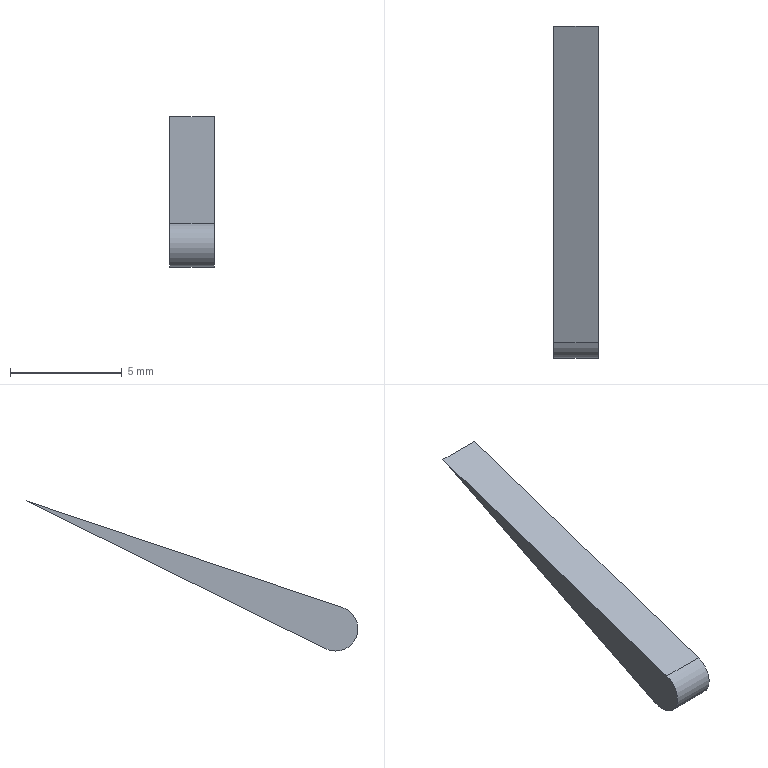Component | NX | CLOCK1 | 1 solid | 5 faces | box 2 x 14.86 x 6.73 mm | volume 33 mm3 | plane 4 | cylinder 1 | commonest cylinder face diameters 2 x1
STEP:
#1=CARTESIAN_POINT('',(0.,0.,0.));
#2=DIRECTION('',(0.,0.,1.));
#3=DIRECTION('',(1.,0.,0.));
#4=AXIS2_PLACEMENT_3D('',#1,#2,#3);
#5=CARTESIAN_POINT('',(-152.42,280.938,31.419));
#6=VERTEX_POINT('',#5);
#7=CARTESIAN_POINT('',(-152.42,281.7,29.575));
#8=VERTEX_POINT('',#7);
#9=CARTESIAN_POINT('',(-152.42,281.257,30.472));
#10=DIRECTION('',(1.,0.,0.));
#11=DIRECTION('',(0.,0.9242,0.3818));
#12=AXIS2_PLACEMENT_3D('',#9,#10,#11);
#13=CIRCLE('',#12,1.);
#14=CARTESIAN_POINT('',(-150.42,281.257,30.472));
#15=DIRECTION('',(-1.,0.,0.));
#16=DIRECTION('',(0.,-0.9242,-0.3818));
#17=AXIS2_PLACEMENT_3D('',#14,#15,#16);
#18=CYLINDRICAL_SURFACE('',#17,1.);
#19=CARTESIAN_POINT('',(9.425,2.));
#20=DIRECTION('',(-1.,0.));
#21=VECTOR('',#20,1.);
#22=LINE('',#19,#21);
#23=(GEOMETRIC_REPRESENTATION_CONTEXT(2)PARAMETRIC_REPRESENTATION_CONTEXT()REPRESENTATION_CONTEXT('',''));
#24=DEFINITIONAL_REPRESENTATION('',(#22),#23);
#25=PCURVE('',#18,#24);
#26=CARTESIAN_POINT('',(-152.42,281.257,30.472));
#27=DIRECTION('',(1.,0.,0.));
#28=DIRECTION('',(0.,0.9242,0.3818));
#29=AXIS2_PLACEMENT_3D('',#26,#27,#28);
#30=PLANE('',#29);
#31=CARTESIAN_POINT('',(0.,0.));
#32=DIRECTION('',(1.,0.));
#33=AXIS2_PLACEMENT_2D('',#31,#32);
#34=CIRCLE('',#33,1.);
#35=(GEOMETRIC_REPRESENTATION_CONTEXT(2)PARAMETRIC_REPRESENTATION_CONTEXT()REPRESENTATION_CONTEXT('',''));
#36=DEFINITIONAL_REPRESENTATION('',(#34),#35);
#37=PCURVE('',#30,#36);
#38=SURFACE_CURVE('',#13,(#25,#37),.PCURVE_S1.);
#39=EDGE_CURVE('',#6,#8,#38,.T.);
#40=ORIENTED_EDGE('',*,*,#39,.T.);
#41=CARTESIAN_POINT('',(-150.42,281.7,29.575));
#42=VERTEX_POINT('',#41);
#43=CARTESIAN_POINT('',(-150.42,281.7,29.575));
#44=DIRECTION('',(-1.,0.,0.));
#45=VECTOR('',#44,1.);
#46=LINE('',#43,#45);
#47=CARTESIAN_POINT('',(4.646,0.));
#48=DIRECTION('',(0.,1.));
#49=VECTOR('',#48,1.);
#50=LINE('',#47,#49);
#51=(GEOMETRIC_REPRESENTATION_CONTEXT(2)PARAMETRIC_REPRESENTATION_CONTEXT()REPRESENTATION_CONTEXT('',''));
#52=DEFINITIONAL_REPRESENTATION('',(#50),#51);
#53=PCURVE('',#18,#52);
#54=CARTESIAN_POINT('',(-150.42,281.7,29.575));
#55=DIRECTION('',(0.,-0.4426,0.8967));
#56=DIRECTION('',(0.,-0.8967,-0.4426));
#57=AXIS2_PLACEMENT_3D('',#54,#55,#56);
#58=PLANE('',#57);
#59=CARTESIAN_POINT('',(0.,0.));
#60=DIRECTION('',(0.,-1.));
#61=VECTOR('',#60,1.);
#62=LINE('',#59,#61);
#63=(GEOMETRIC_REPRESENTATION_CONTEXT(2)PARAMETRIC_REPRESENTATION_CONTEXT()REPRESENTATION_CONTEXT('',''));
#64=DEFINITIONAL_REPRESENTATION('',(#62),#63);
#65=PCURVE('',#58,#64);
#66=SURFACE_CURVE('',#46,(#53,#65),.PCURVE_S1.);
#67=EDGE_CURVE('',#42,#8,#66,.T.);
#68=ORIENTED_EDGE('',*,*,#67,.F.);
#69=CARTESIAN_POINT('',(-150.42,280.938,31.419));
#70=VERTEX_POINT('',#69);
#71=CARTESIAN_POINT('',(-150.42,281.257,30.472));
#72=DIRECTION('',(1.,0.,0.));
#73=DIRECTION('',(0.,0.9242,0.3818));
#74=AXIS2_PLACEMENT_3D('',#71,#72,#73);
#75=CIRCLE('',#74,1.);
#76=CARTESIAN_POINT('',(9.425,0.));
#77=DIRECTION('',(-1.,0.));
#78=VECTOR('',#77,1.);
#79=LINE('',#76,#78);
#80=(GEOMETRIC_REPRESENTATION_CONTEXT(2)PARAMETRIC_REPRESENTATION_CONTEXT()REPRESENTATION_CONTEXT('',''));
#81=DEFINITIONAL_REPRESENTATION('',(#79),#80);
#82=PCURVE('',#18,#81);
#83=CARTESIAN_POINT('',(-150.42,281.257,30.472));
#84=DIRECTION('',(1.,0.,0.));
#85=DIRECTION('',(0.,0.9242,0.3818));
#86=AXIS2_PLACEMENT_3D('',#83,#84,#85);
#87=PLANE('',#86);
#88=CARTESIAN_POINT('',(0.,0.));
#89=DIRECTION('',(1.,0.));
#90=AXIS2_PLACEMENT_2D('',#88,#89);
#91=CIRCLE('',#90,1.);
#92=(GEOMETRIC_REPRESENTATION_CONTEXT(2)PARAMETRIC_REPRESENTATION_CONTEXT()REPRESENTATION_CONTEXT('',''));
#93=DEFINITIONAL_REPRESENTATION('',(#91),#92);
#94=PCURVE('',#87,#93);
#95=SURFACE_CURVE('',#75,(#82,#94),.PCURVE_S1.);
#96=EDGE_CURVE('',#70,#42,#95,.T.);
#97=ORIENTED_EDGE('',*,*,#96,.F.);
#98=CARTESIAN_POINT('',(-150.42,280.938,31.419));
#99=DIRECTION('',(-1.,0.,0.));
#100=VECTOR('',#99,1.);
#101=LINE('',#98,#100);
#102=CARTESIAN_POINT('',(7.921,0.));
#103=DIRECTION('',(0.,1.));
#104=VECTOR('',#103,1.);
#105=LINE('',#102,#104);
#106=(GEOMETRIC_REPRESENTATION_CONTEXT(2)PARAMETRIC_REPRESENTATION_CONTEXT()REPRESENTATION_CONTEXT('',''));
#107=DEFINITIONAL_REPRESENTATION('',(#105),#106);
#108=PCURVE('',#18,#107);
#109=CARTESIAN_POINT('',(-150.42,295.12,36.199));
#110=DIRECTION('',(0.,0.3194,-0.9476));
#111=DIRECTION('',(0.,0.9476,0.3194));
#112=AXIS2_PLACEMENT_3D('',#109,#110,#111);
#113=PLANE('',#112);
#114=CARTESIAN_POINT('',(-14.967,0.));
#115=DIRECTION('',(0.,-1.));
#116=VECTOR('',#115,1.);
#117=LINE('',#114,#116);
#118=(GEOMETRIC_REPRESENTATION_CONTEXT(2)PARAMETRIC_REPRESENTATION_CONTEXT()REPRESENTATION_CONTEXT('',''));
#119=DEFINITIONAL_REPRESENTATION('',(#117),#118);
#120=PCURVE('',#113,#119);
#121=SURFACE_CURVE('',#101,(#108,#120),.PCURVE_S1.);
#122=EDGE_CURVE('',#70,#6,#121,.T.);
#123=ORIENTED_EDGE('',*,*,#122,.T.);
#124=EDGE_LOOP('',(#40,#68,#97,#123));
#125=FACE_BOUND('',#124,.T.);
#126=ADVANCED_FACE('',(#125),#18,.T.);
#127=CARTESIAN_POINT('',(-152.42,295.12,36.199));
#128=VERTEX_POINT('',#127);
#129=CARTESIAN_POINT('',(-152.42,281.7,29.575));
#130=DIRECTION('',(0.,0.8967,0.4426));
#131=VECTOR('',#130,1.);
#132=LINE('',#129,#131);
#133=CARTESIAN_POINT('',(0.,-2.));
#134=DIRECTION('',(-1.,0.));
#135=VECTOR('',#134,1.);
#136=LINE('',#133,#135);
#137=(GEOMETRIC_REPRESENTATION_CONTEXT(2)PARAMETRIC_REPRESENTATION_CONTEXT()REPRESENTATION_CONTEXT('',''));
#138=DEFINITIONAL_REPRESENTATION('',(#136),#137);
#139=PCURVE('',#58,#138);
#140=CARTESIAN_POINT('',(0.06667,-0.9978));
#141=DIRECTION('',(0.9978,0.06667));
#142=VECTOR('',#141,1.);
#143=LINE('',#140,#142);
#144=(GEOMETRIC_REPRESENTATION_CONTEXT(2)PARAMETRIC_REPRESENTATION_CONTEXT()REPRESENTATION_CONTEXT('',''));
#145=DEFINITIONAL_REPRESENTATION('',(#143),#144);
#146=PCURVE('',#30,#145);
#147=SURFACE_CURVE('',#132,(#139,#146),.PCURVE_S1.);
#148=EDGE_CURVE('',#8,#128,#147,.T.);
#149=ORIENTED_EDGE('',*,*,#148,.T.);
#150=CARTESIAN_POINT('',(-150.42,295.12,36.199));
#151=VERTEX_POINT('',#150);
#152=CARTESIAN_POINT('',(-150.42,295.12,36.199));
#153=DIRECTION('',(-1.,0.,0.));
#154=VECTOR('',#153,1.);
#155=LINE('',#152,#154);
#156=CARTESIAN_POINT('',(-14.967,0.));
#157=DIRECTION('',(0.,-1.));
#158=VECTOR('',#157,1.);
#159=LINE('',#156,#158);
#160=(GEOMETRIC_REPRESENTATION_CONTEXT(2)PARAMETRIC_REPRESENTATION_CONTEXT()REPRESENTATION_CONTEXT('',''));
#161=DEFINITIONAL_REPRESENTATION('',(#159),#160);
#162=PCURVE('',#58,#161);
#163=CARTESIAN_POINT('',(0.,0.));
#164=DIRECTION('',(0.,-1.));
#165=VECTOR('',#164,1.);
#166=LINE('',#163,#165);
#167=(GEOMETRIC_REPRESENTATION_CONTEXT(2)PARAMETRIC_REPRESENTATION_CONTEXT()REPRESENTATION_CONTEXT('',''));
#168=DEFINITIONAL_REPRESENTATION('',(#166),#167);
#169=PCURVE('',#113,#168);
#170=SURFACE_CURVE('',#155,(#162,#169),.PCURVE_S1.);
#171=EDGE_CURVE('',#151,#128,#170,.T.);
#172=ORIENTED_EDGE('',*,*,#171,.F.);
#173=CARTESIAN_POINT('',(-150.42,281.7,29.575));
#174=DIRECTION('',(0.,0.8967,0.4426));
#175=VECTOR('',#174,1.);
#176=LINE('',#173,#175);
#177=CARTESIAN_POINT('',(0.,0.));
#178=DIRECTION('',(-1.,0.));
#179=VECTOR('',#178,1.);
#180=LINE('',#177,#179);
#181=(GEOMETRIC_REPRESENTATION_CONTEXT(2)PARAMETRIC_REPRESENTATION_CONTEXT()REPRESENTATION_CONTEXT('',''));
#182=DEFINITIONAL_REPRESENTATION('',(#180),#181);
#183=PCURVE('',#58,#182);
#184=CARTESIAN_POINT('',(0.06667,-0.9978));
#185=DIRECTION('',(0.9978,0.06667));
#186=VECTOR('',#185,1.);
#187=LINE('',#184,#186);
#188=(GEOMETRIC_REPRESENTATION_CONTEXT(2)PARAMETRIC_REPRESENTATION_CONTEXT()REPRESENTATION_CONTEXT('',''));
#189=DEFINITIONAL_REPRESENTATION('',(#187),#188);
#190=PCURVE('',#87,#189);
#191=SURFACE_CURVE('',#176,(#183,#190),.PCURVE_S1.);
#192=EDGE_CURVE('',#42,#151,#191,.T.);
#193=ORIENTED_EDGE('',*,*,#192,.F.);
#194=ORIENTED_EDGE('',*,*,#67,.T.);
#195=EDGE_LOOP('',(#149,#172,#193,#194));
#196=FACE_BOUND('',#195,.T.);
#197=ADVANCED_FACE('',(#196),#58,.F.);
#198=CARTESIAN_POINT('',(-152.42,295.12,36.199));
#199=DIRECTION('',(0.,-0.9476,-0.3194));
#200=VECTOR('',#199,1.);
#201=LINE('',#198,#200);
#202=CARTESIAN_POINT('',(0.,-2.));
#203=DIRECTION('',(-1.,0.));
#204=VECTOR('',#203,1.);
#205=LINE('',#202,#204);
#206=(GEOMETRIC_REPRESENTATION_CONTEXT(2)PARAMETRIC_REPRESENTATION_CONTEXT()REPRESENTATION_CONTEXT('',''));
#207=DEFINITIONAL_REPRESENTATION('',(#205),#206);
#208=PCURVE('',#113,#207);
#209=CARTESIAN_POINT('',(15.,0.));
#210=DIRECTION('',(-0.9978,0.06667));
#211=VECTOR('',#210,1.);
#212=LINE('',#209,#211);
#213=(GEOMETRIC_REPRESENTATION_CONTEXT(2)PARAMETRIC_REPRESENTATION_CONTEXT()REPRESENTATION_CONTEXT('',''));
#214=DEFINITIONAL_REPRESENTATION('',(#212),#213);
#215=PCURVE('',#30,#214);
#216=SURFACE_CURVE('',#201,(#208,#215),.PCURVE_S1.);
#217=EDGE_CURVE('',#128,#6,#216,.T.);
#218=ORIENTED_EDGE('',*,*,#217,.T.);
#219=ORIENTED_EDGE('',*,*,#122,.F.);
#220=CARTESIAN_POINT('',(-150.42,295.12,36.199));
#221=DIRECTION('',(0.,-0.9476,-0.3194));
#222=VECTOR('',#221,1.);
#223=LINE('',#220,#222);
#224=CARTESIAN_POINT('',(0.,0.));
#225=DIRECTION('',(-1.,0.));
#226=VECTOR('',#225,1.);
#227=LINE('',#224,#226);
#228=(GEOMETRIC_REPRESENTATION_CONTEXT(2)PARAMETRIC_REPRESENTATION_CONTEXT()REPRESENTATION_CONTEXT('',''));
#229=DEFINITIONAL_REPRESENTATION('',(#227),#228);
#230=PCURVE('',#113,#229);
#231=CARTESIAN_POINT('',(15.,0.));
#232=DIRECTION('',(-0.9978,0.06667));
#233=VECTOR('',#232,1.);
#234=LINE('',#231,#233);
#235=(GEOMETRIC_REPRESENTATION_CONTEXT(2)PARAMETRIC_REPRESENTATION_CONTEXT()REPRESENTATION_CONTEXT('',''));
#236=DEFINITIONAL_REPRESENTATION('',(#234),#235);
#237=PCURVE('',#87,#236);
#238=SURFACE_CURVE('',#223,(#230,#237),.PCURVE_S1.);
#239=EDGE_CURVE('',#151,#70,#238,.T.);
#240=ORIENTED_EDGE('',*,*,#239,.F.);
#241=ORIENTED_EDGE('',*,*,#171,.T.);
#242=EDGE_LOOP('',(#218,#219,#240,#241));
#243=FACE_BOUND('',#242,.T.);
#244=ADVANCED_FACE('',(#243),#113,.F.);
#245=ORIENTED_EDGE('',*,*,#96,.T.);
#246=ORIENTED_EDGE('',*,*,#192,.T.);
#247=ORIENTED_EDGE('',*,*,#239,.T.);
#248=EDGE_LOOP('',(#245,#246,#247));
#249=FACE_BOUND('',#248,.T.);
#250=ADVANCED_FACE('',(#249),#87,.T.);
#251=ORIENTED_EDGE('',*,*,#39,.F.);
#252=ORIENTED_EDGE('',*,*,#217,.F.);
#253=ORIENTED_EDGE('',*,*,#148,.F.);
#254=EDGE_LOOP('',(#251,#252,#253));
#255=FACE_BOUND('',#254,.T.);
#256=ADVANCED_FACE('',(#255),#30,.F.);
#257=CLOSED_SHELL('',(#126,#197,#244,#250,#256));
#258=MANIFOLD_SOLID_BREP('',#257);
#259=(LENGTH_UNIT()NAMED_UNIT(*)SI_UNIT(.MILLI.,.METRE.));
#260=UNCERTAINTY_MEASURE_WITH_UNIT(LENGTH_MEASURE(0.0000001),#259,'','');
#261=(NAMED_UNIT(*)PLANE_ANGLE_UNIT()SI_UNIT($,.RADIAN.));
#262=(NAMED_UNIT(*)SI_UNIT($,.STERADIAN.)SOLID_ANGLE_UNIT());
#263=(GEOMETRIC_REPRESENTATION_CONTEXT(3)GLOBAL_UNCERTAINTY_ASSIGNED_CONTEXT((#260))GLOBAL_UNIT_ASSIGNED_CONTEXT((#259,#261,#262))REPRESENTATION_CONTEXT('',''));
#264=ADVANCED_BREP_SHAPE_REPRESENTATION('',(#4,#258),#263);